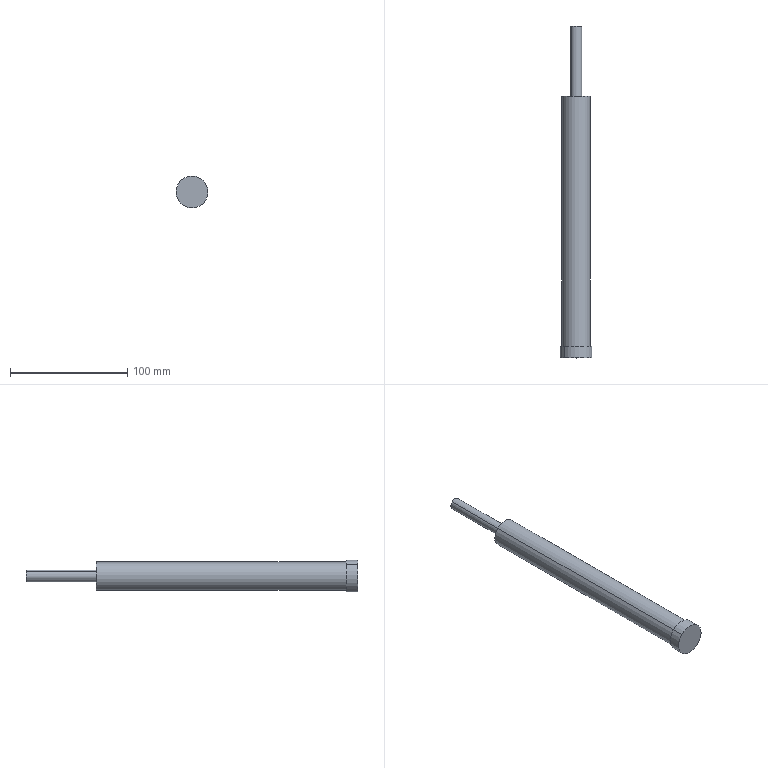Component | SolidWorks | AdjustableHydraulicBufferHR60-1 | 1 solid | 10 faces | box 27.3 x 283.5 x 27.3 mm | volume 107151 mm3 | cylinder 6 | plane 4 | commonest cylinder face diameters 10 x2 24 x2 27.3 x2
build123d program:
from build123d import *

# Parameters (mm, degrees)
SKETCH1_R           = 13.65
BOSS_EXTRUDE1_DEPTH = 10
SKETCH2_R           = 12
BOSS_EXTRUDE2_DEPTH = 213.5
SKETCH3_R           = 5
BOSS_EXTRUDE3_DEPTH = 60


with BuildPart() as part:
    # Sketch1 → Boss-Extrude1 (new body)
    with BuildSketch(Plane(origin=(0, 0, 0), x_dir=(1, 0, 0), z_dir=(0, 1, 0))):
        with Locations(Location((0, 0, 0), (0, 0, 270))):
            Circle(SKETCH1_R)
    extrude(amount=BOSS_EXTRUDE1_DEPTH)

    # Sketch2 → Boss-Extrude2 (add)
    with BuildSketch(Plane(origin=(0, 10, 0), x_dir=(1, 0, 0), z_dir=(0, 1, 0))):
        with Locations(Location((0, 0, 0), (0, 0, 270))):
            Circle(SKETCH2_R)
    extrude(amount=BOSS_EXTRUDE2_DEPTH)

    # Sketch3 → Boss-Extrude3 (add)
    with BuildSketch(Plane(origin=(0, 223.5, 0), x_dir=(1, 0, 0), z_dir=(0, 1, 0))):
        with Locations(Location((0, 0, 0), (0, 0, 270))):
            Circle(SKETCH3_R)
    extrude(amount=BOSS_EXTRUDE3_DEPTH)


solid = part.part

# Placed as in the assembly
solid = solid.moved(Location((-115.446, -379.666, 991.405), (0, 0, 0)))
STEP:
#1=COLOUR_RGB('',0.7922,0.8196,0.9333);
#2=FILL_AREA_STYLE_COLOUR('',#1);
#3=FILL_AREA_STYLE('',(#2));
#4=SURFACE_STYLE_FILL_AREA(#3);
#5=SURFACE_SIDE_STYLE('',(#4));
#6=SURFACE_STYLE_USAGE(.BOTH.,#5);
#7=PRESENTATION_STYLE_ASSIGNMENT((#6));
#8=CARTESIAN_POINT('',(-4.406,-3.786,38.892));
#9=VERTEX_POINT('',#8);
#10=CARTESIAN_POINT('',(-4.684,-3.786,39.171));
#11=VERTEX_POINT('',#10);
#12=CARTESIAN_POINT('',(-4.545,-3.786,39.032));
#13=DIRECTION('',(-0.,1.,0.));
#14=DIRECTION('',(0.7071,0.,-0.7071));
#15=AXIS2_PLACEMENT_3D('',#12,#13,#14);
#16=CIRCLE('',#15,0.1969);
#17=EDGE_CURVE('',#9,#11,#16,.T.);
#18=ORIENTED_EDGE('',*,*,#17,.F.);
#19=CARTESIAN_POINT('',(-4.406,-6.148,38.892));
#20=VERTEX_POINT('',#19);
#21=CARTESIAN_POINT('',(-4.406,-3.786,38.892));
#22=DIRECTION('',(0.,-1.,-0.));
#23=VECTOR('',#22,39.37);
#24=LINE('',#21,#23);
#25=EDGE_CURVE('',#9,#20,#24,.T.);
#26=ORIENTED_EDGE('',*,*,#25,.T.);
#27=CARTESIAN_POINT('',(-4.684,-6.148,39.171));
#28=VERTEX_POINT('',#27);
#29=CARTESIAN_POINT('',(-4.545,-6.148,39.032));
#30=DIRECTION('',(-0.,1.,0.));
#31=DIRECTION('',(0.7071,0.,-0.7071));
#32=AXIS2_PLACEMENT_3D('',#29,#30,#31);
#33=CIRCLE('',#32,0.1969);
#34=EDGE_CURVE('',#20,#28,#33,.T.);
#35=ORIENTED_EDGE('',*,*,#34,.T.);
#36=CARTESIAN_POINT('',(-4.684,-3.786,39.171));
#37=DIRECTION('',(0.,-1.,-0.));
#38=VECTOR('',#37,39.37);
#39=LINE('',#36,#38);
#40=EDGE_CURVE('',#11,#28,#39,.T.);
#41=ORIENTED_EDGE('',*,*,#40,.F.);
#42=EDGE_LOOP('',(#18,#26,#35,#41));
#43=FACE_OUTER_BOUND('',#42,.T.);
#44=CARTESIAN_POINT('',(-4.545,-3.786,39.032));
#45=DIRECTION('',(0.,-1.,-0.));
#46=DIRECTION('',(-0.7071,0.,0.7071));
#47=AXIS2_PLACEMENT_3D('',#44,#45,#46);
#48=CYLINDRICAL_SURFACE('',#47,0.1969);
#49=ADVANCED_FACE('',(#43),#48,.T.);
#50=CARTESIAN_POINT('',(-4.211,-6.148,38.698));
#51=VERTEX_POINT('',#50);
#52=CARTESIAN_POINT('',(-4.879,-6.148,39.366));
#53=VERTEX_POINT('',#52);
#54=CARTESIAN_POINT('',(-4.545,-6.148,39.032));
#55=DIRECTION('',(-0.,1.,0.));
#56=DIRECTION('',(0.7071,0.,-0.7071));
#57=AXIS2_PLACEMENT_3D('',#54,#55,#56);
#58=CIRCLE('',#57,0.4724);
#59=EDGE_CURVE('',#51,#53,#58,.T.);
#60=ORIENTED_EDGE('',*,*,#59,.F.);
#61=CARTESIAN_POINT('',(-4.211,-14.554,38.698));
#62=VERTEX_POINT('',#61);
#63=CARTESIAN_POINT('',(-4.211,-6.148,38.698));
#64=DIRECTION('',(0.,-1.,-0.));
#65=VECTOR('',#64,39.37);
#66=LINE('',#63,#65);
#67=EDGE_CURVE('',#51,#62,#66,.T.);
#68=ORIENTED_EDGE('',*,*,#67,.T.);
#69=CARTESIAN_POINT('',(-4.879,-14.554,39.366));
#70=VERTEX_POINT('',#69);
#71=CARTESIAN_POINT('',(-4.545,-14.554,39.032));
#72=DIRECTION('',(-0.,1.,0.));
#73=DIRECTION('',(0.7071,0.,-0.7071));
#74=AXIS2_PLACEMENT_3D('',#71,#72,#73);
#75=CIRCLE('',#74,0.4724);
#76=EDGE_CURVE('',#62,#70,#75,.T.);
#77=ORIENTED_EDGE('',*,*,#76,.T.);
#78=CARTESIAN_POINT('',(-4.879,-6.148,39.366));
#79=DIRECTION('',(0.,-1.,-0.));
#80=VECTOR('',#79,39.37);
#81=LINE('',#78,#80);
#82=EDGE_CURVE('',#53,#70,#81,.T.);
#83=ORIENTED_EDGE('',*,*,#82,.F.);
#84=EDGE_LOOP('',(#60,#68,#77,#83));
#85=FACE_OUTER_BOUND('',#84,.T.);
#86=CARTESIAN_POINT('',(-4.545,-6.148,39.032));
#87=DIRECTION('',(0.,-1.,-0.));
#88=DIRECTION('',(-0.7071,0.,0.7071));
#89=AXIS2_PLACEMENT_3D('',#86,#87,#88);
#90=CYLINDRICAL_SURFACE('',#89,0.4724);
#91=ADVANCED_FACE('',(#85),#90,.T.);
#92=CARTESIAN_POINT('',(-4.165,-14.554,38.652));
#93=VERTEX_POINT('',#92);
#94=CARTESIAN_POINT('',(-4.925,-14.554,39.412));
#95=VERTEX_POINT('',#94);
#96=CARTESIAN_POINT('',(-4.545,-14.554,39.032));
#97=DIRECTION('',(-0.,1.,0.));
#98=DIRECTION('',(0.7071,0.,-0.7071));
#99=AXIS2_PLACEMENT_3D('',#96,#97,#98);
#100=CIRCLE('',#99,0.5374);
#101=EDGE_CURVE('',#93,#95,#100,.T.);
#102=ORIENTED_EDGE('',*,*,#101,.F.);
#103=CARTESIAN_POINT('',(-4.165,-14.947,38.652));
#104=VERTEX_POINT('',#103);
#105=CARTESIAN_POINT('',(-4.165,-14.554,38.652));
#106=DIRECTION('',(0.,-1.,-0.));
#107=VECTOR('',#106,39.37);
#108=LINE('',#105,#107);
#109=EDGE_CURVE('',#93,#104,#108,.T.);
#110=ORIENTED_EDGE('',*,*,#109,.T.);
#111=CARTESIAN_POINT('',(-4.925,-14.947,39.412));
#112=VERTEX_POINT('',#111);
#113=CARTESIAN_POINT('',(-4.545,-14.947,39.032));
#114=DIRECTION('',(-0.,1.,0.));
#115=DIRECTION('',(0.7071,0.,-0.7071));
#116=AXIS2_PLACEMENT_3D('',#113,#114,#115);
#117=CIRCLE('',#116,0.5374);
#118=EDGE_CURVE('',#104,#112,#117,.T.);
#119=ORIENTED_EDGE('',*,*,#118,.T.);
#120=CARTESIAN_POINT('',(-4.925,-14.554,39.412));
#121=DIRECTION('',(0.,-1.,-0.));
#122=VECTOR('',#121,39.37);
#123=LINE('',#120,#122);
#124=EDGE_CURVE('',#95,#112,#123,.T.);
#125=ORIENTED_EDGE('',*,*,#124,.F.);
#126=EDGE_LOOP('',(#102,#110,#119,#125));
#127=FACE_OUTER_BOUND('',#126,.T.);
#128=CARTESIAN_POINT('',(-4.545,-14.554,39.032));
#129=DIRECTION('',(0.,-1.,-0.));
#130=DIRECTION('',(-0.7071,0.,0.7071));
#131=AXIS2_PLACEMENT_3D('',#128,#129,#130);
#132=CYLINDRICAL_SURFACE('',#131,0.5374);
#133=ADVANCED_FACE('',(#127),#132,.T.);
#134=ORIENTED_EDGE('',*,*,#109,.F.);
#135=CARTESIAN_POINT('',(-4.545,-14.554,39.032));
#136=DIRECTION('',(-0.,1.,0.));
#137=DIRECTION('',(0.7071,0.,-0.7071));
#138=AXIS2_PLACEMENT_3D('',#135,#136,#137);
#139=CIRCLE('',#138,0.5374);
#140=EDGE_CURVE('',#95,#93,#139,.T.);
#141=ORIENTED_EDGE('',*,*,#140,.F.);
#142=ORIENTED_EDGE('',*,*,#124,.T.);
#143=CARTESIAN_POINT('',(-4.545,-14.947,39.032));
#144=DIRECTION('',(-0.,1.,0.));
#145=DIRECTION('',(0.7071,0.,-0.7071));
#146=AXIS2_PLACEMENT_3D('',#143,#144,#145);
#147=CIRCLE('',#146,0.5374);
#148=EDGE_CURVE('',#112,#104,#147,.T.);
#149=ORIENTED_EDGE('',*,*,#148,.T.);
#150=EDGE_LOOP('',(#134,#141,#142,#149));
#151=FACE_OUTER_BOUND('',#150,.T.);
#152=CARTESIAN_POINT('',(-4.545,-14.554,39.032));
#153=DIRECTION('',(0.,-1.,-0.));
#154=DIRECTION('',(-0.7071,0.,0.7071));
#155=AXIS2_PLACEMENT_3D('',#152,#153,#154);
#156=CYLINDRICAL_SURFACE('',#155,0.5374);
#157=ADVANCED_FACE('',(#151),#156,.T.);
#158=CARTESIAN_POINT('',(-4.545,-14.554,39.032));
#159=DIRECTION('',(-0.,1.,0.));
#160=DIRECTION('',(0.7071,0.,-0.7071));
#161=AXIS2_PLACEMENT_3D('',#158,#159,#160);
#162=CIRCLE('',#161,0.4724);
#163=EDGE_CURVE('',#70,#62,#162,.T.);
#164=ORIENTED_EDGE('',*,*,#163,.F.);
#165=ORIENTED_EDGE('',*,*,#76,.F.);
#166=EDGE_LOOP('',(#164,#165));
#167=FACE_BOUND('',#166,.T.);
#168=ORIENTED_EDGE('',*,*,#140,.T.);
#169=ORIENTED_EDGE('',*,*,#101,.T.);
#170=EDGE_LOOP('',(#168,#169));
#171=FACE_OUTER_BOUND('',#170,.T.);
#172=CARTESIAN_POINT('',(-4.545,-14.554,39.032));
#173=DIRECTION('',(-0.,1.,0.));
#174=DIRECTION('',(0.7071,0.,-0.7071));
#175=AXIS2_PLACEMENT_3D('',#172,#173,#174);
#176=PLANE('',#175);
#177=ADVANCED_FACE('',(#167,#171),#176,.T.);
#178=ORIENTED_EDGE('',*,*,#148,.F.);
#179=ORIENTED_EDGE('',*,*,#118,.F.);
#180=EDGE_LOOP('',(#178,#179));
#181=FACE_OUTER_BOUND('',#180,.T.);
#182=CARTESIAN_POINT('',(-4.545,-14.947,39.032));
#183=DIRECTION('',(-0.,1.,0.));
#184=DIRECTION('',(0.7071,0.,-0.7071));
#185=AXIS2_PLACEMENT_3D('',#182,#183,#184);
#186=PLANE('',#185);
#187=ADVANCED_FACE('',(#181),#186,.F.);
#188=ORIENTED_EDGE('',*,*,#67,.F.);
#189=CARTESIAN_POINT('',(-4.545,-6.148,39.032));
#190=DIRECTION('',(-0.,1.,0.));
#191=DIRECTION('',(0.7071,0.,-0.7071));
#192=AXIS2_PLACEMENT_3D('',#189,#190,#191);
#193=CIRCLE('',#192,0.4724);
#194=EDGE_CURVE('',#53,#51,#193,.T.);
#195=ORIENTED_EDGE('',*,*,#194,.F.);
#196=ORIENTED_EDGE('',*,*,#82,.T.);
#197=ORIENTED_EDGE('',*,*,#163,.T.);
#198=EDGE_LOOP('',(#188,#195,#196,#197));
#199=FACE_OUTER_BOUND('',#198,.T.);
#200=CARTESIAN_POINT('',(-4.545,-6.148,39.032));
#201=DIRECTION('',(0.,-1.,-0.));
#202=DIRECTION('',(-0.7071,0.,0.7071));
#203=AXIS2_PLACEMENT_3D('',#200,#201,#202);
#204=CYLINDRICAL_SURFACE('',#203,0.4724);
#205=ADVANCED_FACE('',(#199),#204,.T.);
#206=CARTESIAN_POINT('',(-4.545,-6.148,39.032));
#207=DIRECTION('',(-0.,1.,0.));
#208=DIRECTION('',(0.7071,0.,-0.7071));
#209=AXIS2_PLACEMENT_3D('',#206,#207,#208);
#210=CIRCLE('',#209,0.1969);
#211=EDGE_CURVE('',#28,#20,#210,.T.);
#212=ORIENTED_EDGE('',*,*,#211,.F.);
#213=ORIENTED_EDGE('',*,*,#34,.F.);
#214=EDGE_LOOP('',(#212,#213));
#215=FACE_BOUND('',#214,.T.);
#216=ORIENTED_EDGE('',*,*,#194,.T.);
#217=ORIENTED_EDGE('',*,*,#59,.T.);
#218=EDGE_LOOP('',(#216,#217));
#219=FACE_OUTER_BOUND('',#218,.T.);
#220=CARTESIAN_POINT('',(-4.545,-6.148,39.032));
#221=DIRECTION('',(-0.,1.,0.));
#222=DIRECTION('',(0.7071,0.,-0.7071));
#223=AXIS2_PLACEMENT_3D('',#220,#221,#222);
#224=PLANE('',#223);
#225=ADVANCED_FACE('',(#215,#219),#224,.T.);
#226=ORIENTED_EDGE('',*,*,#25,.F.);
#227=CARTESIAN_POINT('',(-4.545,-3.786,39.032));
#228=DIRECTION('',(-0.,1.,0.));
#229=DIRECTION('',(0.7071,0.,-0.7071));
#230=AXIS2_PLACEMENT_3D('',#227,#228,#229);
#231=CIRCLE('',#230,0.1969);
#232=EDGE_CURVE('',#11,#9,#231,.T.);
#233=ORIENTED_EDGE('',*,*,#232,.F.);
#234=ORIENTED_EDGE('',*,*,#40,.T.);
#235=ORIENTED_EDGE('',*,*,#211,.T.);
#236=EDGE_LOOP('',(#226,#233,#234,#235));
#237=FACE_OUTER_BOUND('',#236,.T.);
#238=CARTESIAN_POINT('',(-4.545,-3.786,39.032));
#239=DIRECTION('',(0.,-1.,-0.));
#240=DIRECTION('',(-0.7071,0.,0.7071));
#241=AXIS2_PLACEMENT_3D('',#238,#239,#240);
#242=CYLINDRICAL_SURFACE('',#241,0.1969);
#243=ADVANCED_FACE('',(#237),#242,.T.);
#244=ORIENTED_EDGE('',*,*,#232,.T.);
#245=ORIENTED_EDGE('',*,*,#17,.T.);
#246=EDGE_LOOP('',(#244,#245));
#247=FACE_OUTER_BOUND('',#246,.T.);
#248=CARTESIAN_POINT('',(-4.545,-3.786,39.032));
#249=DIRECTION('',(-0.,1.,0.));
#250=DIRECTION('',(0.7071,0.,-0.7071));
#251=AXIS2_PLACEMENT_3D('',#248,#249,#250);
#252=PLANE('',#251);
#253=ADVANCED_FACE('',(#247),#252,.T.);
#254=CLOSED_SHELL('',(#49,#91,#133,#157,#177,#187,#205,#225,#243,#253));
#255=MANIFOLD_SOLID_BREP('',#254);
#256=STYLED_ITEM('',(#7),#255);
#257=(LENGTH_UNIT()NAMED_UNIT(*)SI_UNIT($,.METRE.));
#258=LENGTH_MEASURE_WITH_UNIT(LENGTH_MEASURE(0.0254),#257);
#259=DIMENSIONAL_EXPONENTS(1.,0.,0.,0.,0.,0.,0.);
#260=(CONVERSION_BASED_UNIT('',#258)LENGTH_UNIT()NAMED_UNIT(#259));
#261=UNCERTAINTY_MEASURE_WITH_UNIT(LENGTH_MEASURE(0.00001),#260,'','');
#262=(NAMED_UNIT(*)PLANE_ANGLE_UNIT()SI_UNIT($,.RADIAN.));
#263=(NAMED_UNIT(*)SI_UNIT($,.STERADIAN.)SOLID_ANGLE_UNIT());
#264=(GEOMETRIC_REPRESENTATION_CONTEXT(3)GLOBAL_UNCERTAINTY_ASSIGNED_CONTEXT((#261))GLOBAL_UNIT_ASSIGNED_CONTEXT((#260,#262,#263))REPRESENTATION_CONTEXT('',''));
#265=MECHANICAL_DESIGN_GEOMETRIC_PRESENTATION_REPRESENTATION('',(#256),#264);
#266=PRESENTATION_LAYER_ASSIGNMENT('','',(#256));
#267=CARTESIAN_POINT('',(0.,0.,0.));
#268=DIRECTION('',(0.,0.,1.));
#269=DIRECTION('',(1.,0.,0.));
#270=AXIS2_PLACEMENT_3D('',#267,#268,#269);
#271=(LENGTH_UNIT()NAMED_UNIT(*)SI_UNIT($,.METRE.));
#272=LENGTH_MEASURE_WITH_UNIT(LENGTH_MEASURE(0.0254),#271);
#273=DIMENSIONAL_EXPONENTS(1.,0.,0.,0.,0.,0.,0.);
#274=(CONVERSION_BASED_UNIT('',#272)LENGTH_UNIT()NAMED_UNIT(#273));
#275=UNCERTAINTY_MEASURE_WITH_UNIT(LENGTH_MEASURE(0.00001),#274,'','');
#276=(NAMED_UNIT(*)PLANE_ANGLE_UNIT()SI_UNIT($,.RADIAN.));
#277=(NAMED_UNIT(*)SI_UNIT($,.STERADIAN.)SOLID_ANGLE_UNIT());
#278=(GEOMETRIC_REPRESENTATION_CONTEXT(3)GLOBAL_UNCERTAINTY_ASSIGNED_CONTEXT((#275))GLOBAL_UNIT_ASSIGNED_CONTEXT((#274,#276,#277))REPRESENTATION_CONTEXT('',''));
#279=ADVANCED_BREP_SHAPE_REPRESENTATION('',(#255,#270),#278);